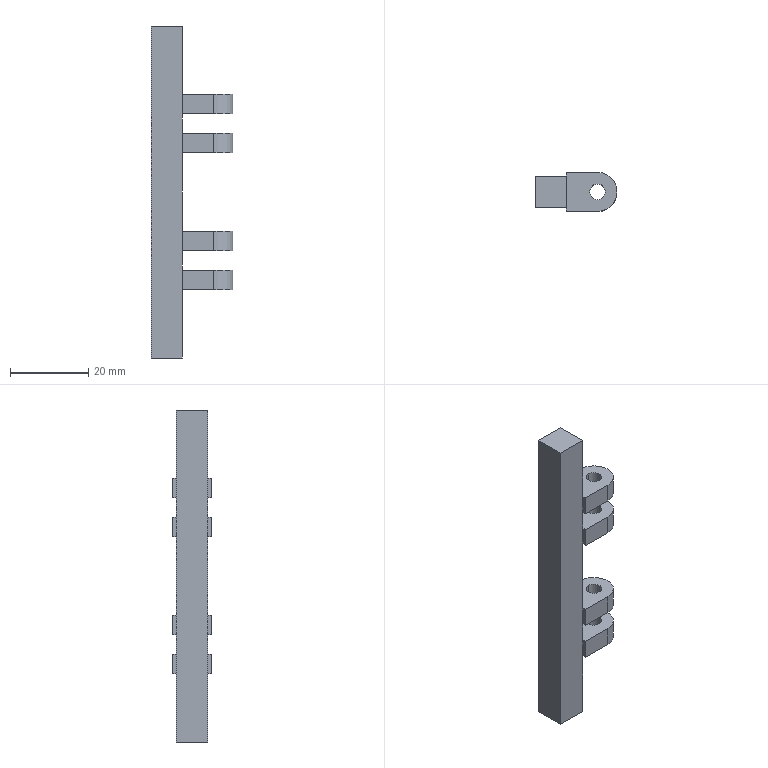Component | SolidWorks | WheelAssembly-1_DamperBase-1 | 1 solid | 46 faces | box 21 x 10 x 85 mm | volume 7574 mm3 | plane 34 | cylinder 12 | commonest cylinder face diameters 4 x8 10 x4
build123d program:
from build123d import *

# Parameters (mm, degrees)
SKETCH1_W               = 8
SKETCH1_H               = 8
BOSS_EXTRUDE1_DEPTH     = 42.5
SKETCH2_R               = 2
BOSS_EXTRUDE2_DEPTH     = 25
CUT_EXTRUDE1_DEPTH      = 47.65
CUT_EXTRUDE1_DEPTH_BACK = 47.65
SKETCH3_W               = 5
SKETCH3_H               = 17.65
SKETCH3_W_2             = 20
SKETCH3_H_2             = 17.022


with BuildPart() as part:
    # Sketch1 → Boss-Extrude1 (new, symmetric)
    with BuildSketch(Plane.XY):
        Rectangle(SKETCH1_W, SKETCH1_H)
    extrude(amount=BOSS_EXTRUDE1_DEPTH, both=True)

    # Sketch2 → Boss-Extrude2 (add, symmetric)
    with BuildSketch(Plane.XY):
        with BuildLine():
            Line((-5, -12), (-5, -4))
            Line((-5, -4), (5, -4))
            Line((5, -4), (5, -12))
            ThreePointArc((5, -12), (0, -17), (-5, -12))
        make_face()
        with Locations((0, -12)):
            Circle(SKETCH2_R, mode=Mode.SUBTRACT)
    extrude(amount=BOSS_EXTRUDE2_DEPTH, both=True)

    # Sketch3 → Cut-Extrude1 (cut, two sides: drawn at the far end of the back side and taken through both)
    with BuildSketch(Plane(origin=(4, 0, 0), x_dir=(0, 0, -1), z_dir=(1, 0, 0)).offset(-CUT_EXTRUDE1_DEPTH_BACK)):
        with Locations((-17.5, -12.825)):
            Rectangle(SKETCH3_W, SKETCH3_H)
        with Locations((17.5, -12.825)):
            Rectangle(SKETCH3_W, SKETCH3_H)
        with Locations((0, -12.511)):
            Rectangle(SKETCH3_W_2, SKETCH3_H_2)
    extrude(amount=CUT_EXTRUDE1_DEPTH + CUT_EXTRUDE1_DEPTH_BACK, mode=Mode.SUBTRACT)


solid = part.part

# Placed as in the assembly
solid = solid.moved(Location((-356, -129, -542.97), (0, 0, 90)))